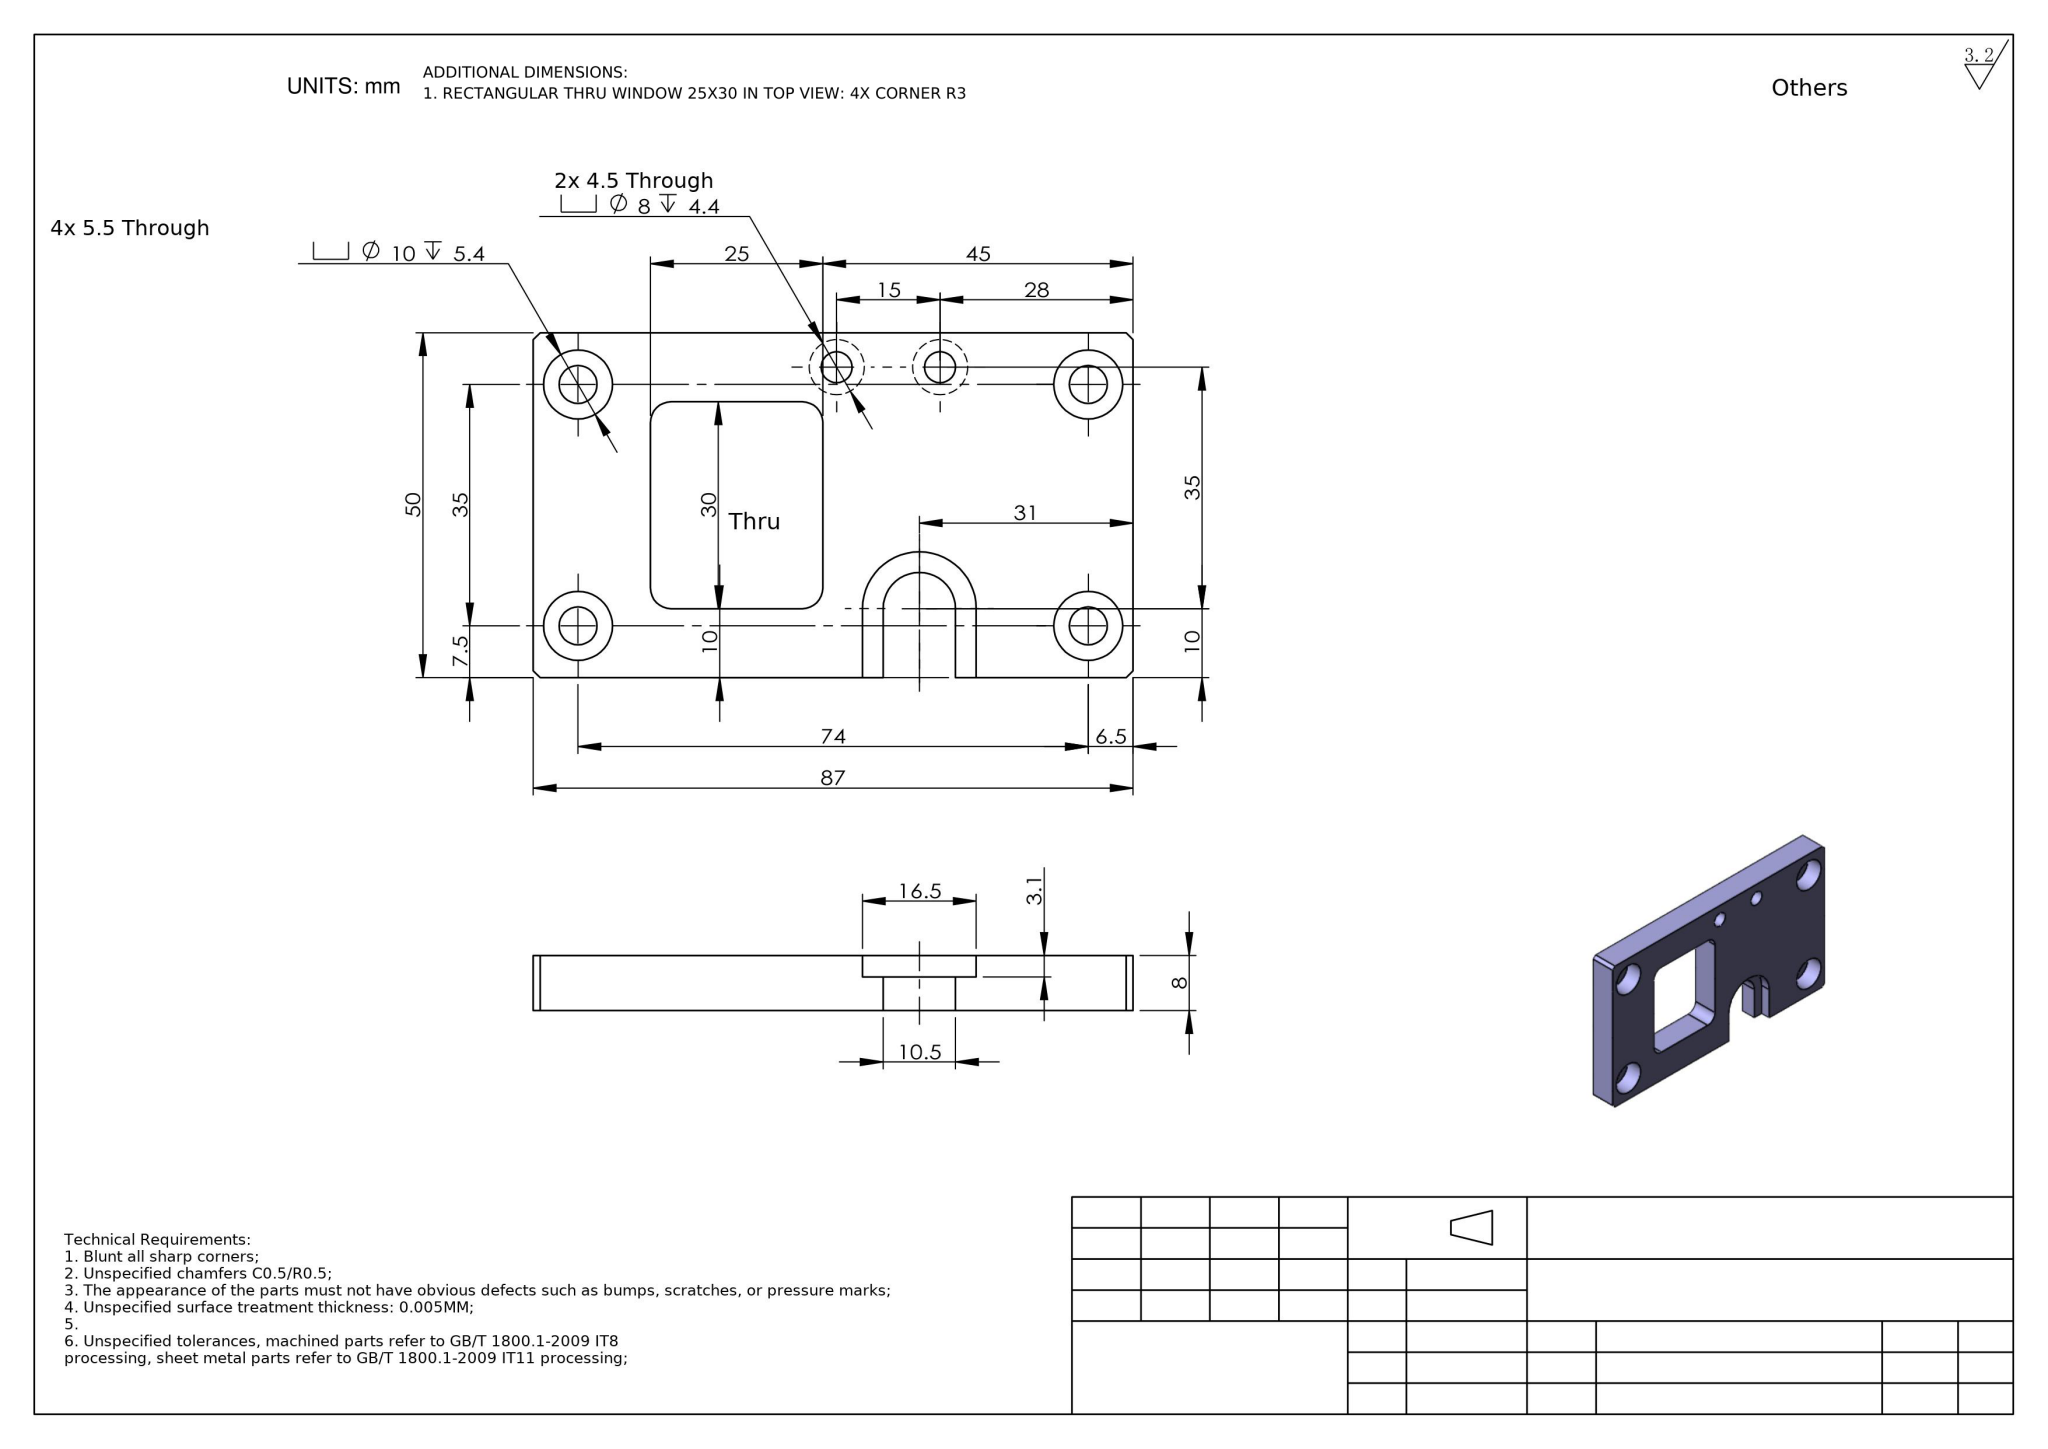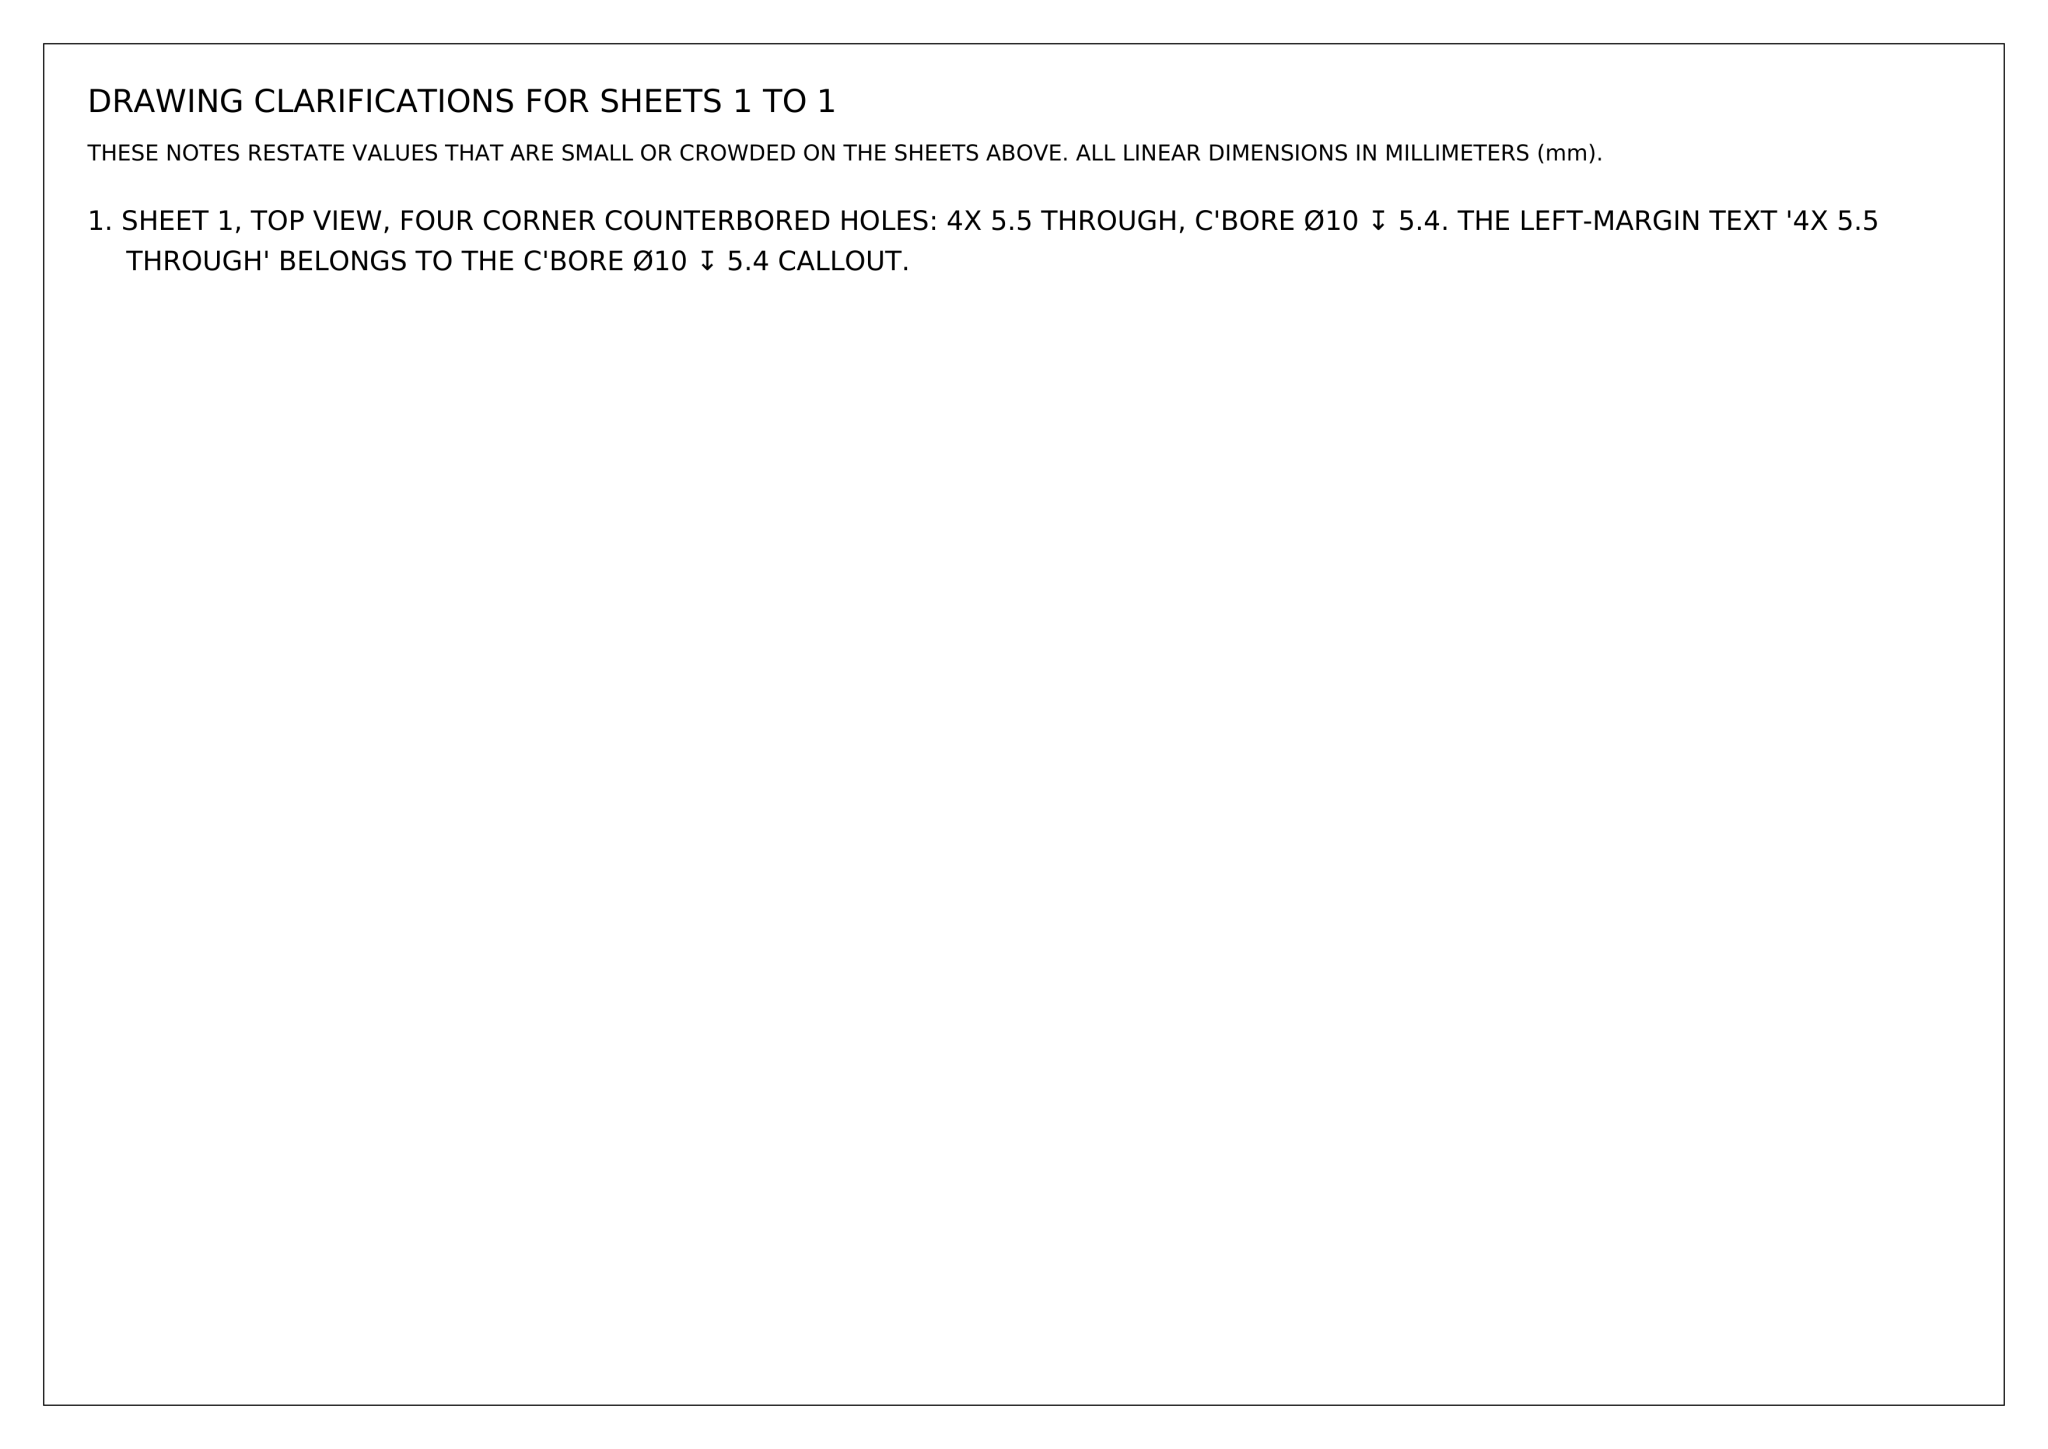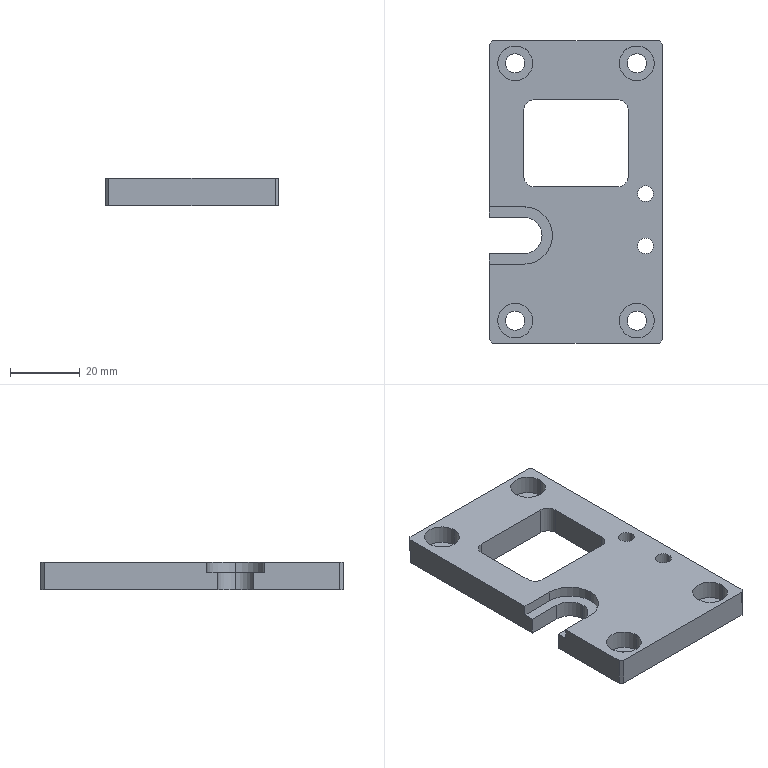Part | NX | mm | 1 solid | 58 faces | box 50 x 87 x 8 mm | volume 24776 mm3 | cylinder 32 | plane 26 | commonest cylinder face diameters 10 x8 5.5 x8 8 x4 4.5 x4 6 x4 16.5 x2 10.5 x2